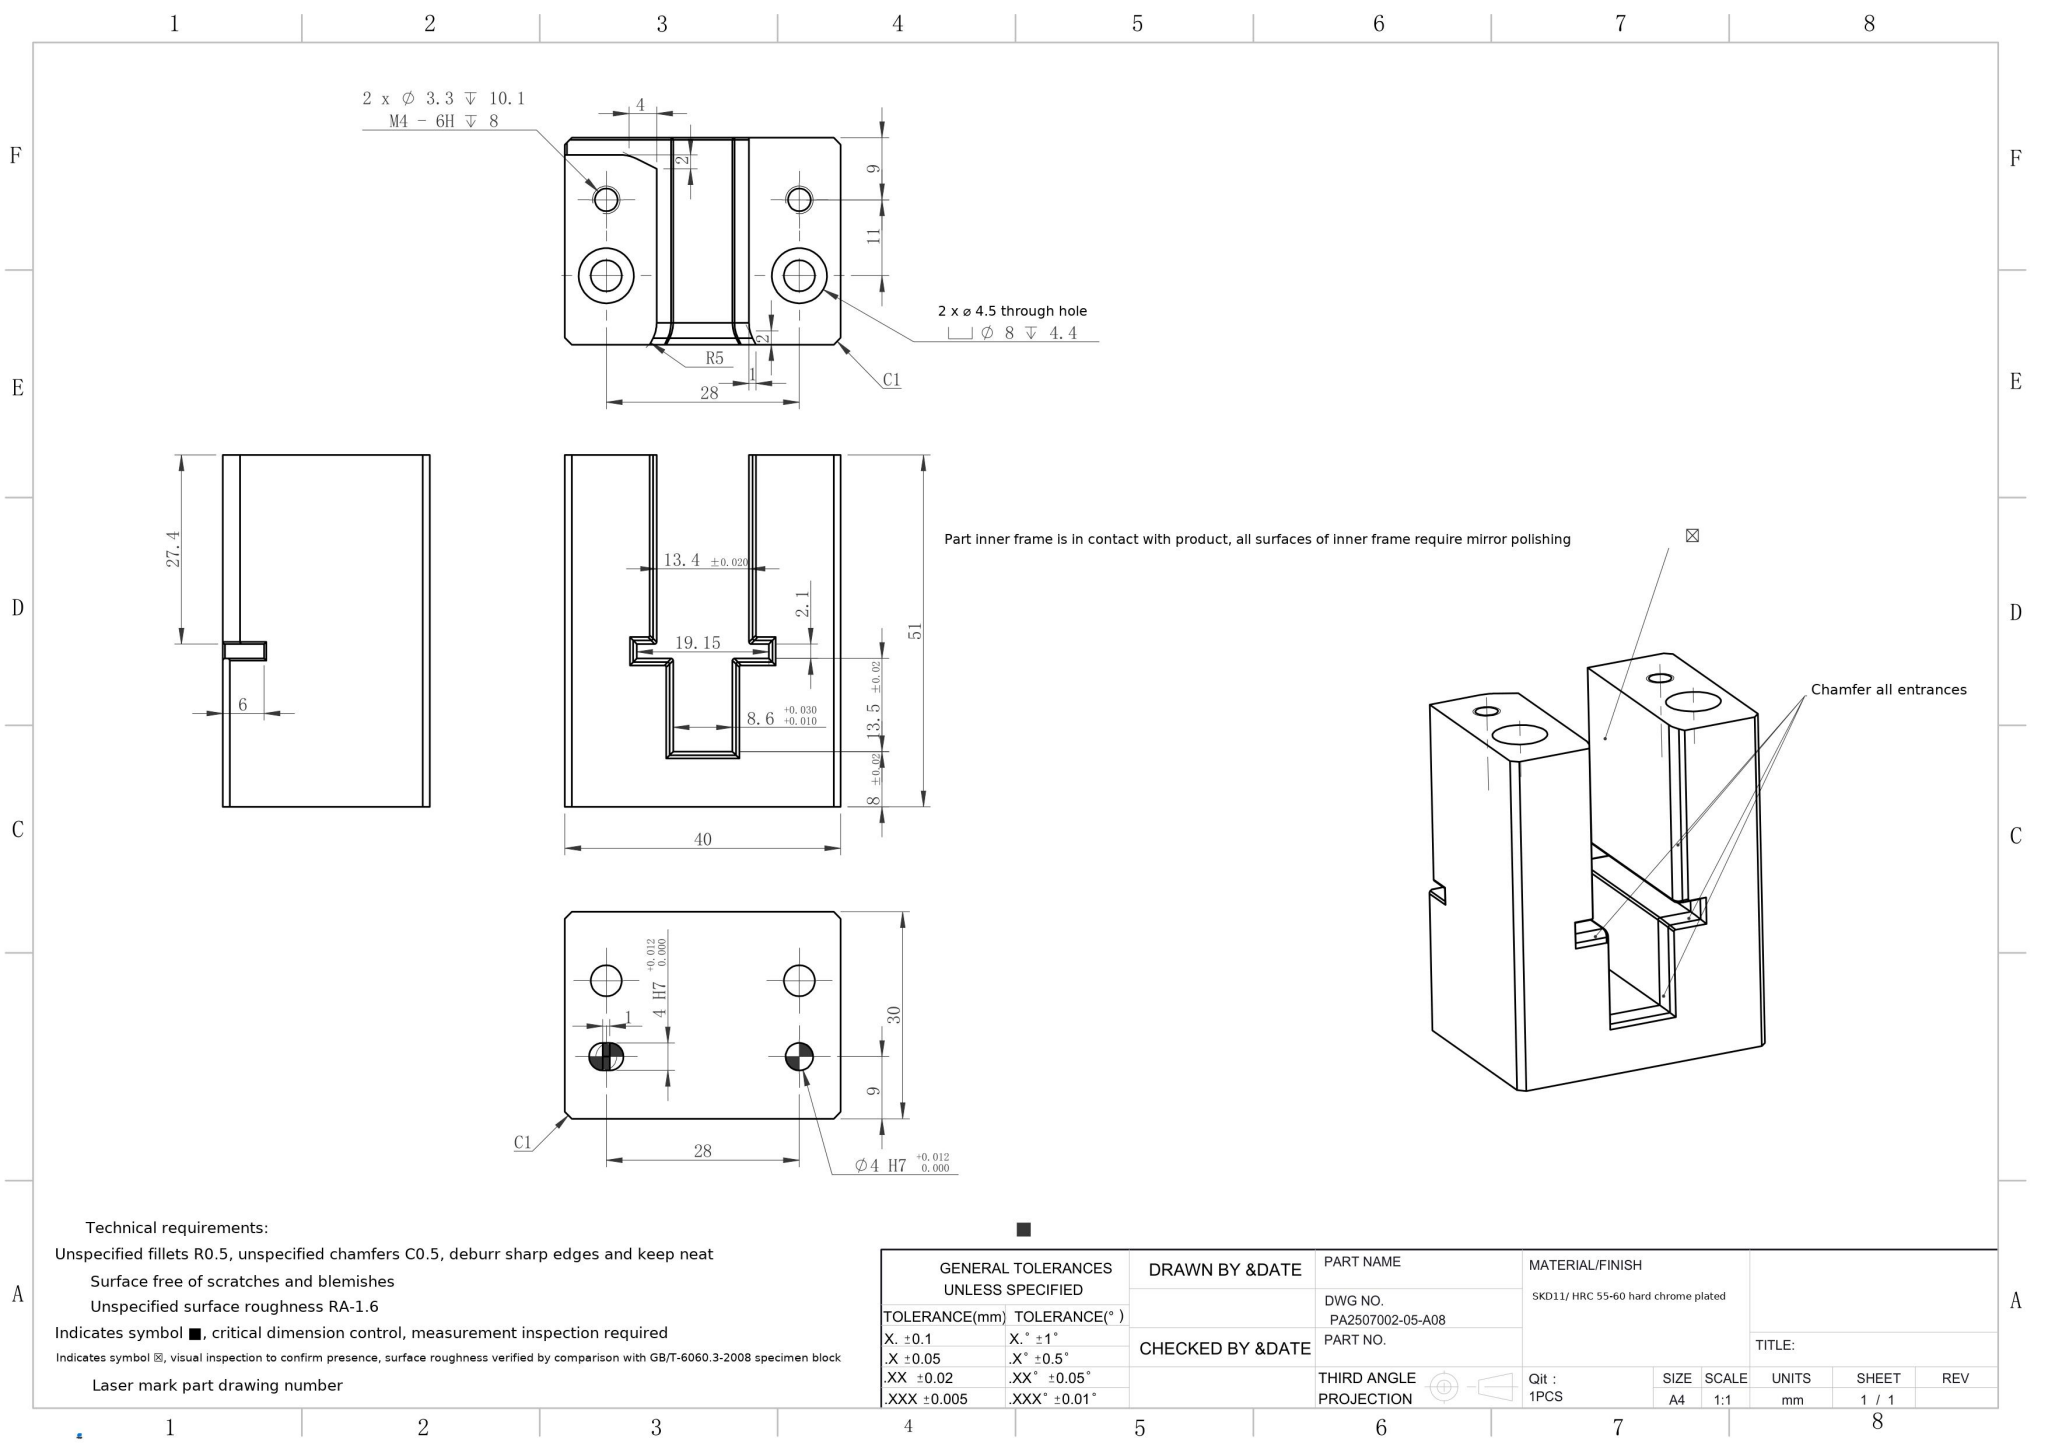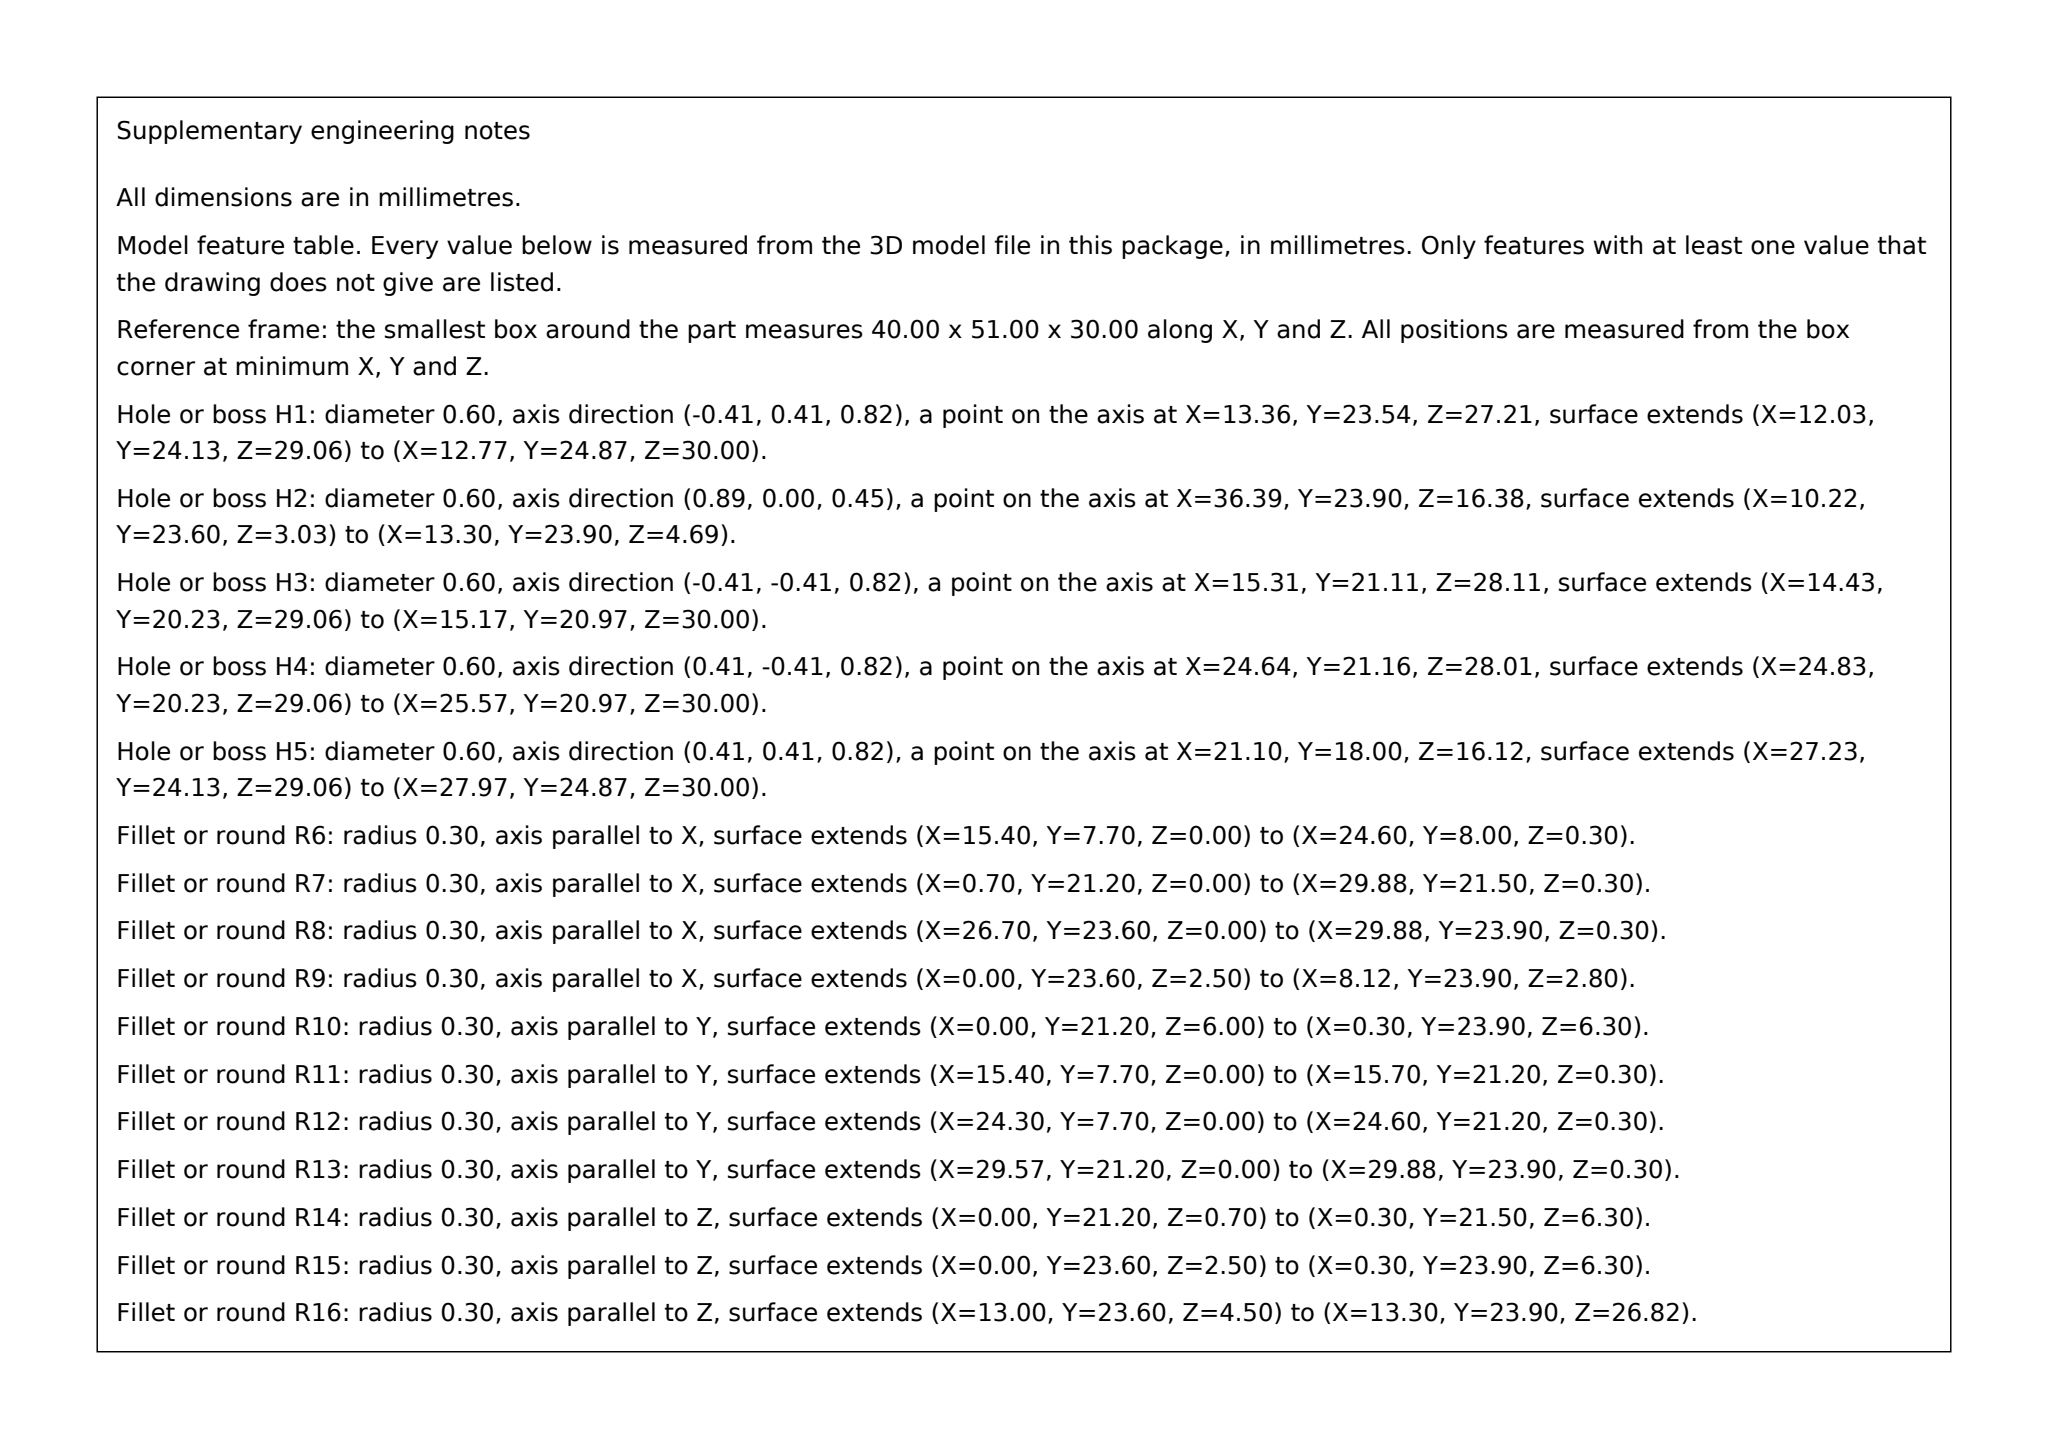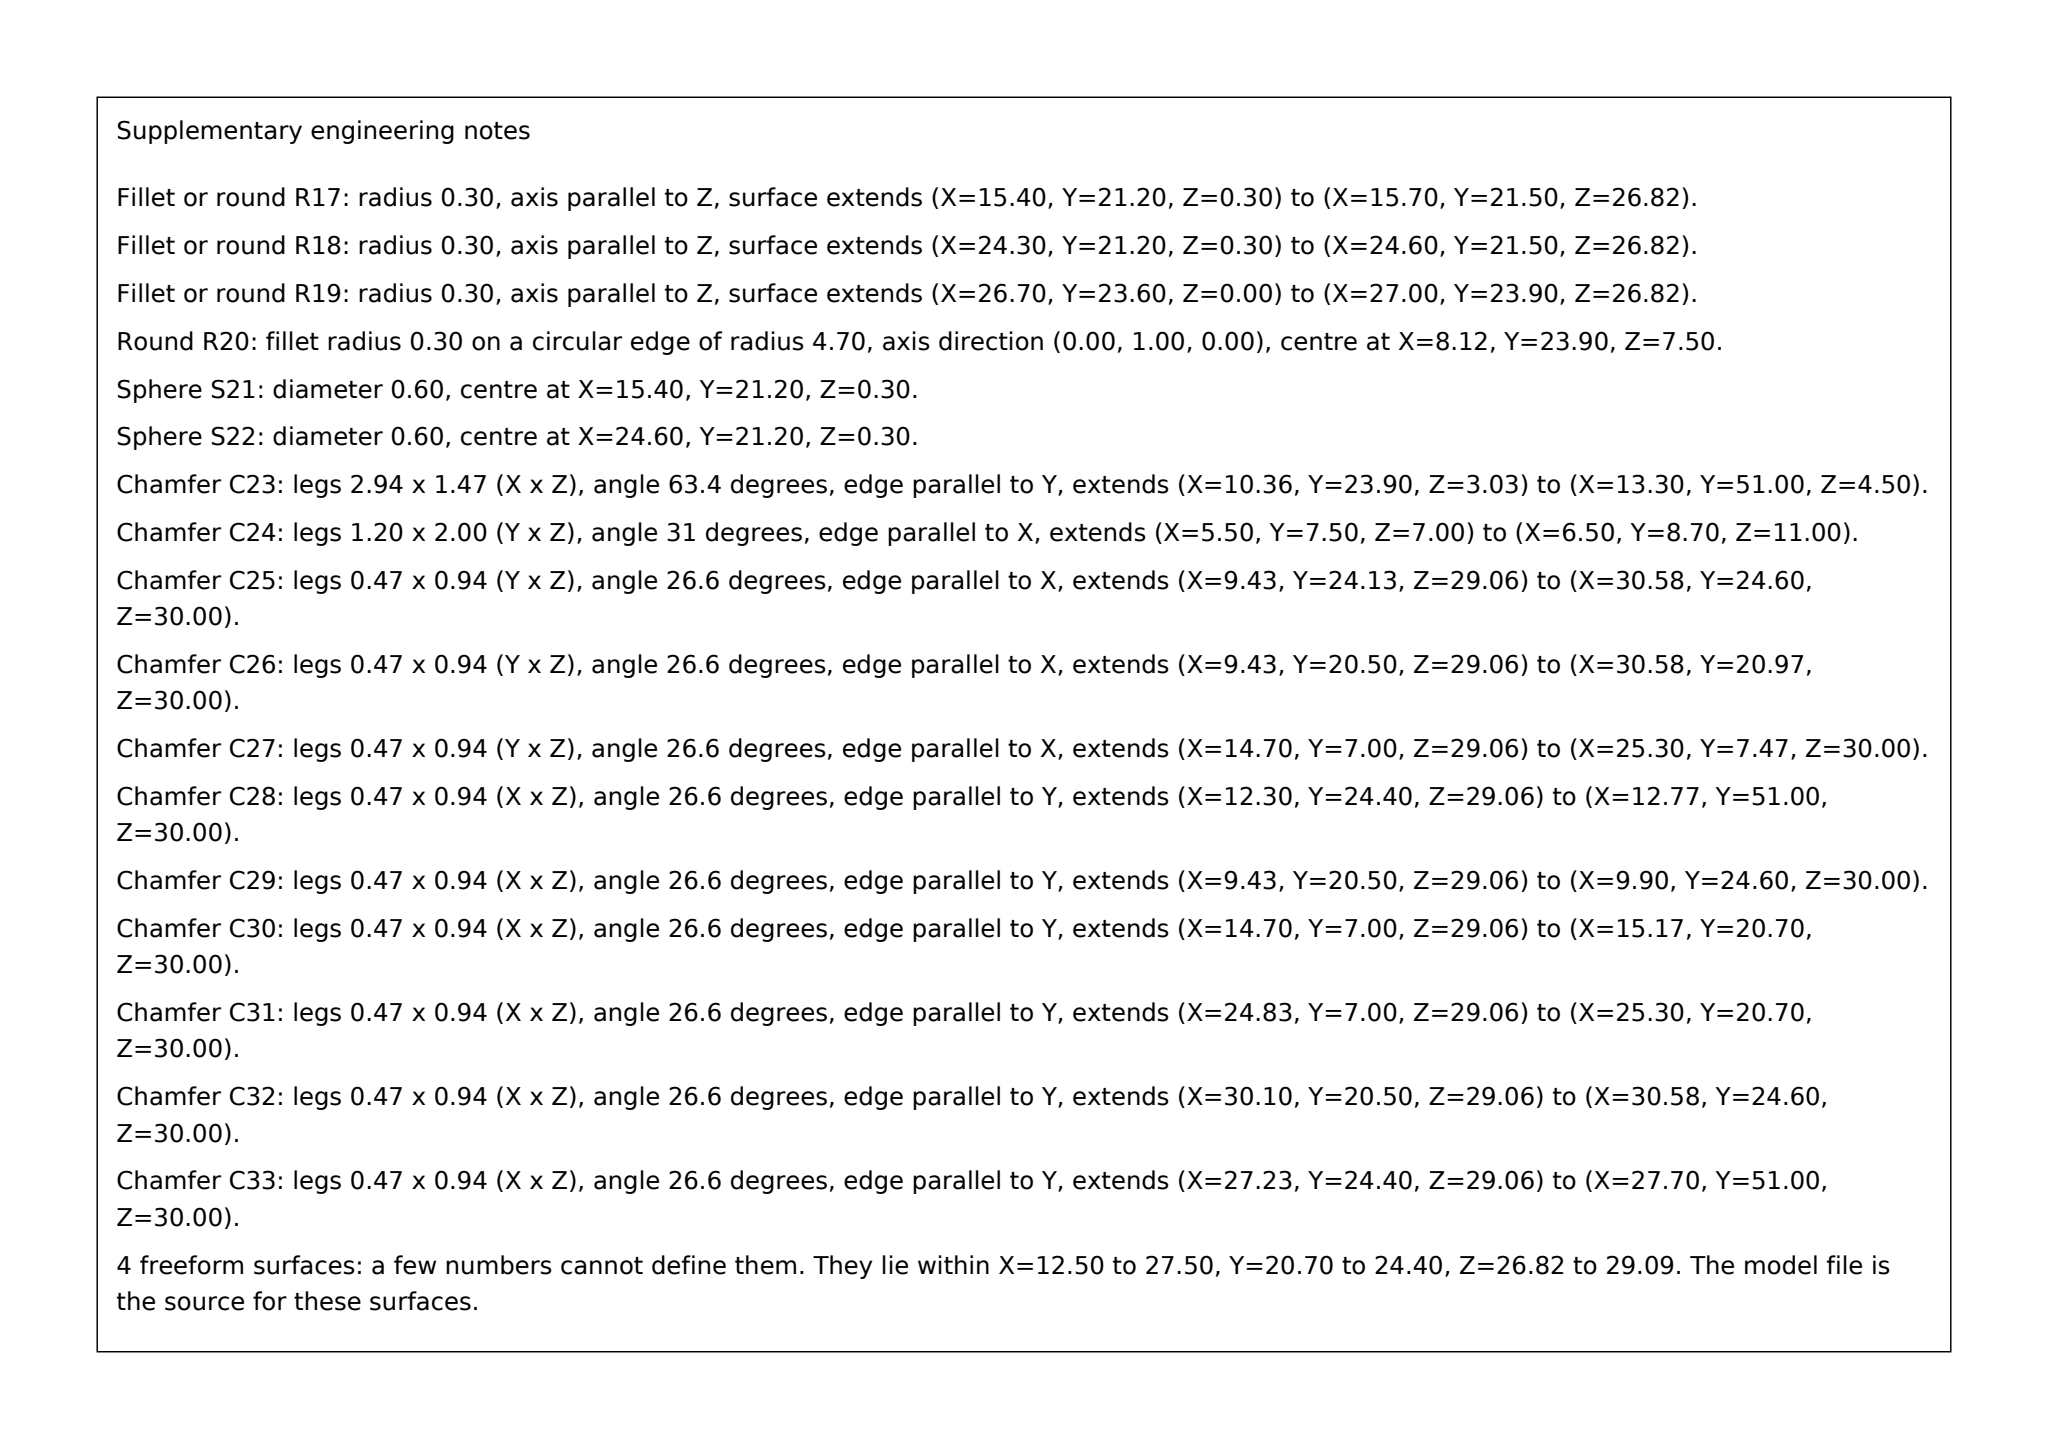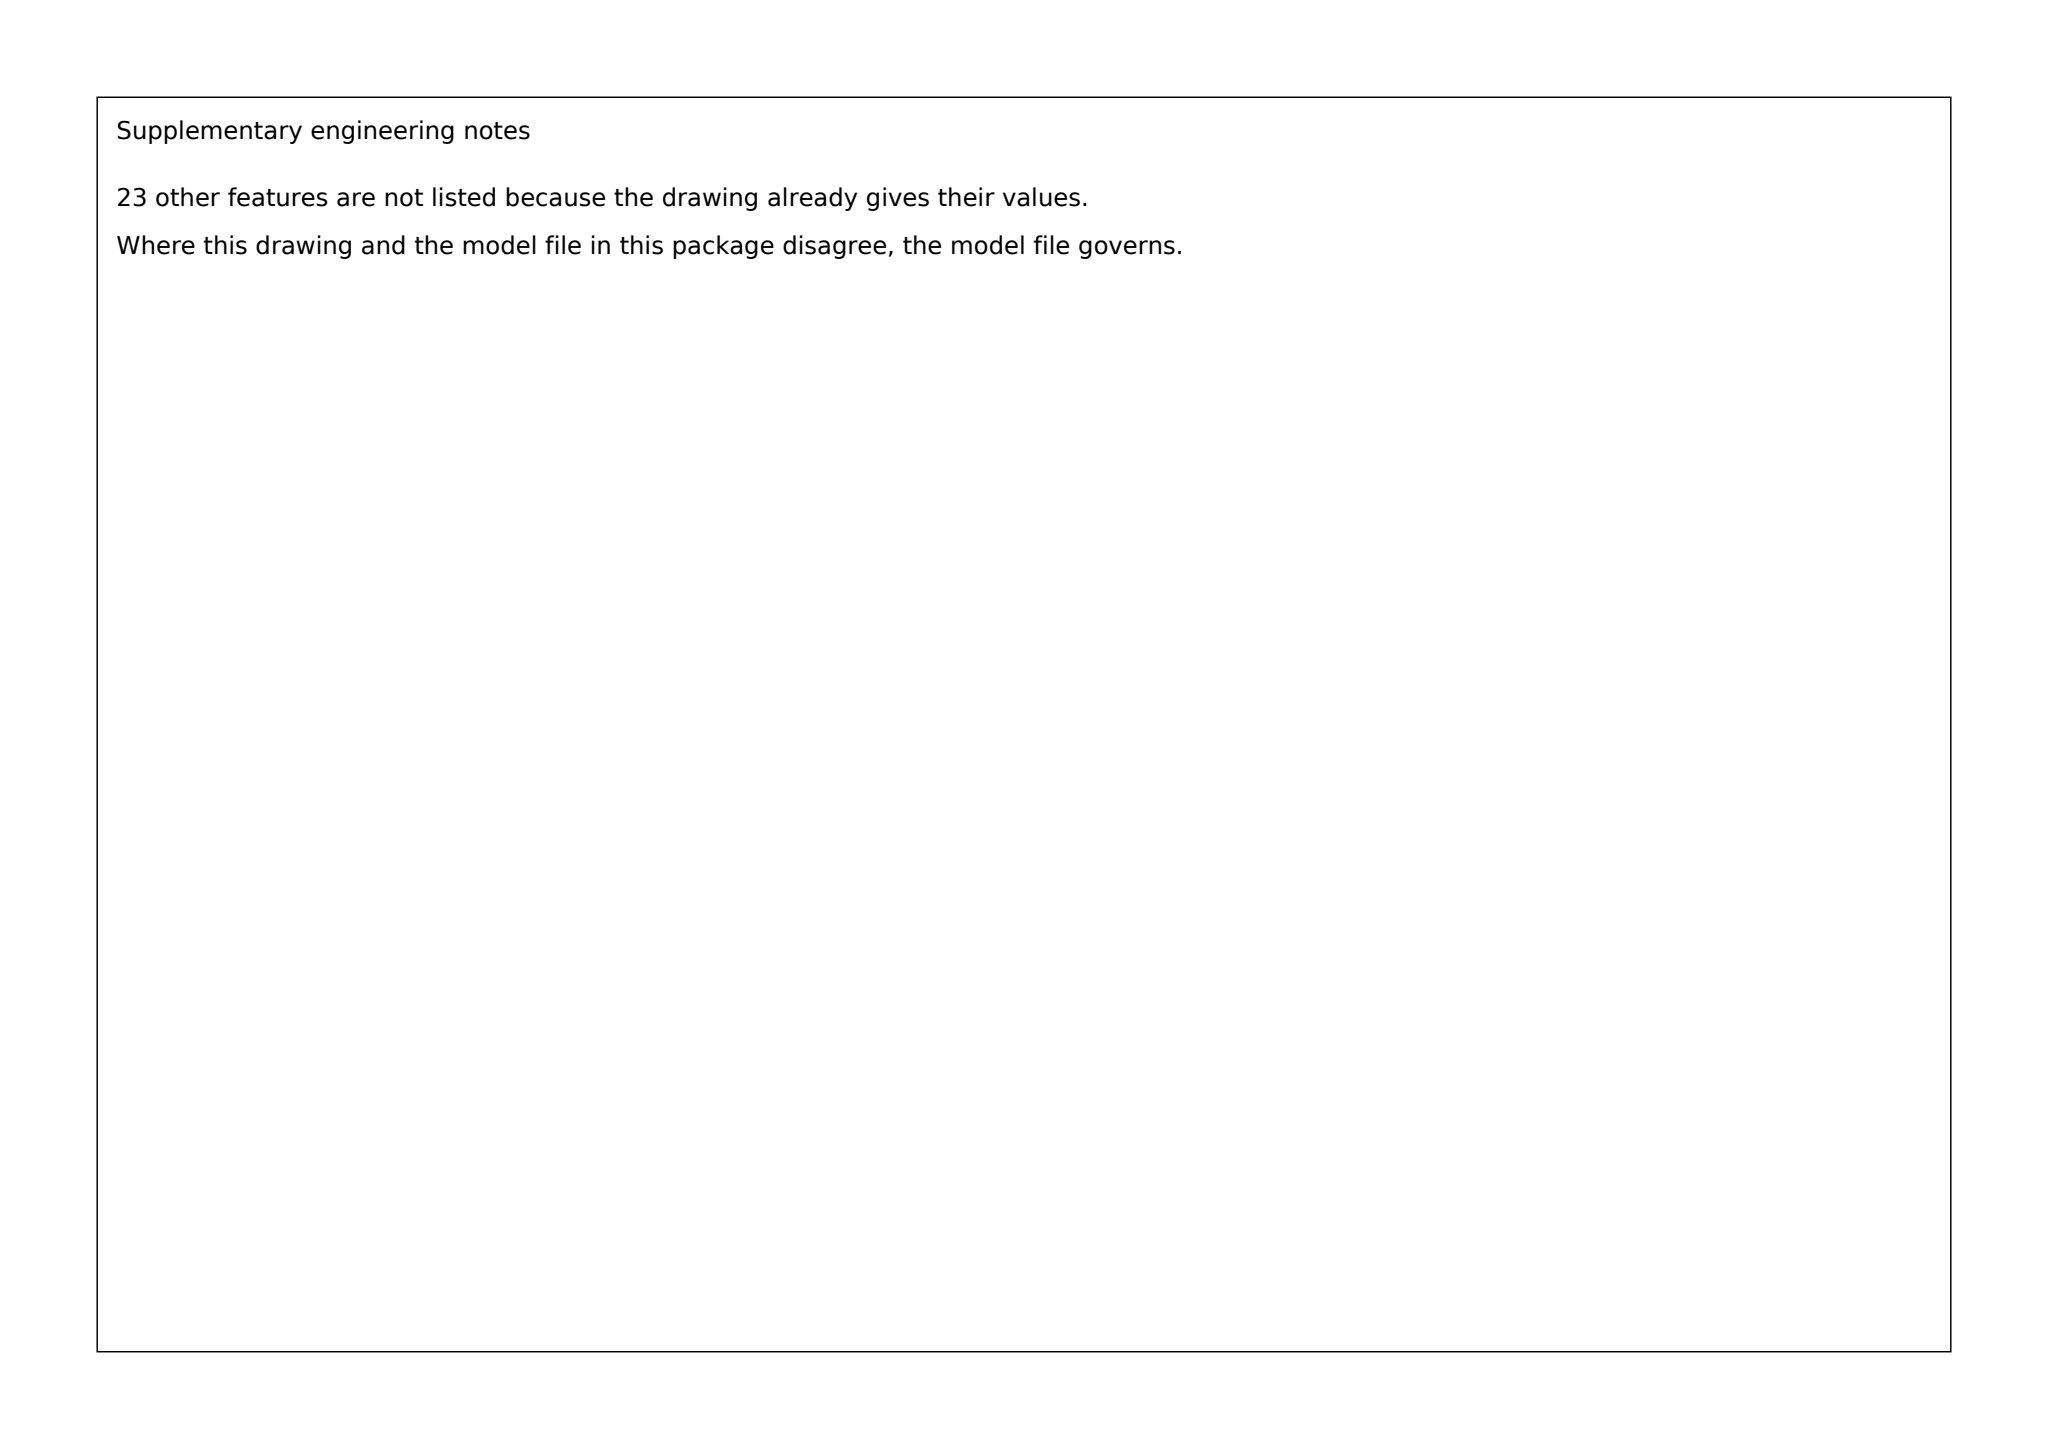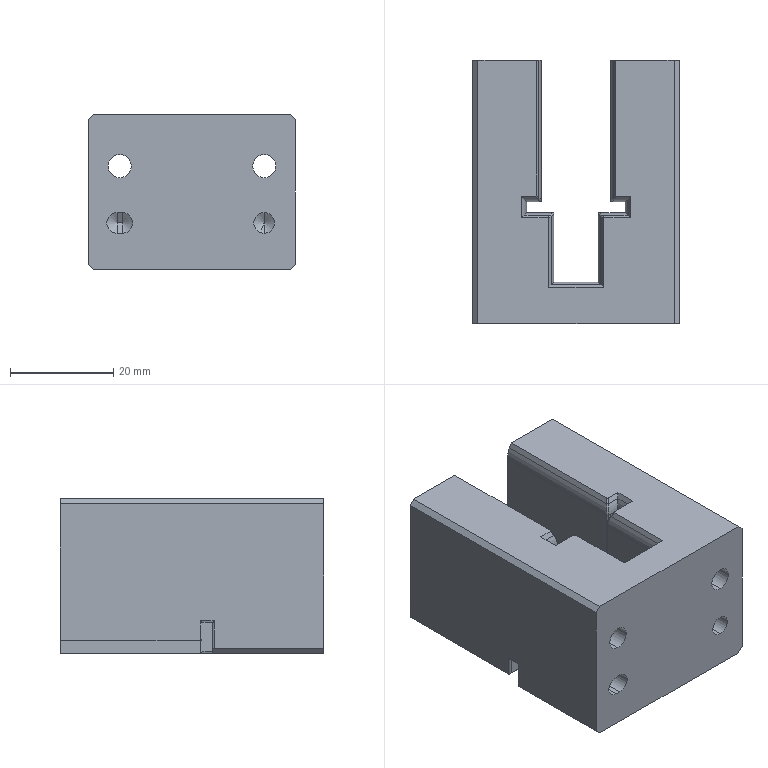Part | SolidWorks | mm | material SKD11/ HRC 55-60 hard chrome plated | 1 solid | 105 faces | box 40 x 51 x 30 mm | volume 41792 mm3 | cylinder 48 | plane 42 | cone 8 | spline 4 | sphere 2 | torus 1 | commonest cylinder face diameters 0.6 x20 10 x12 4 x4 3.3 x4 8 x4 4.5 x4